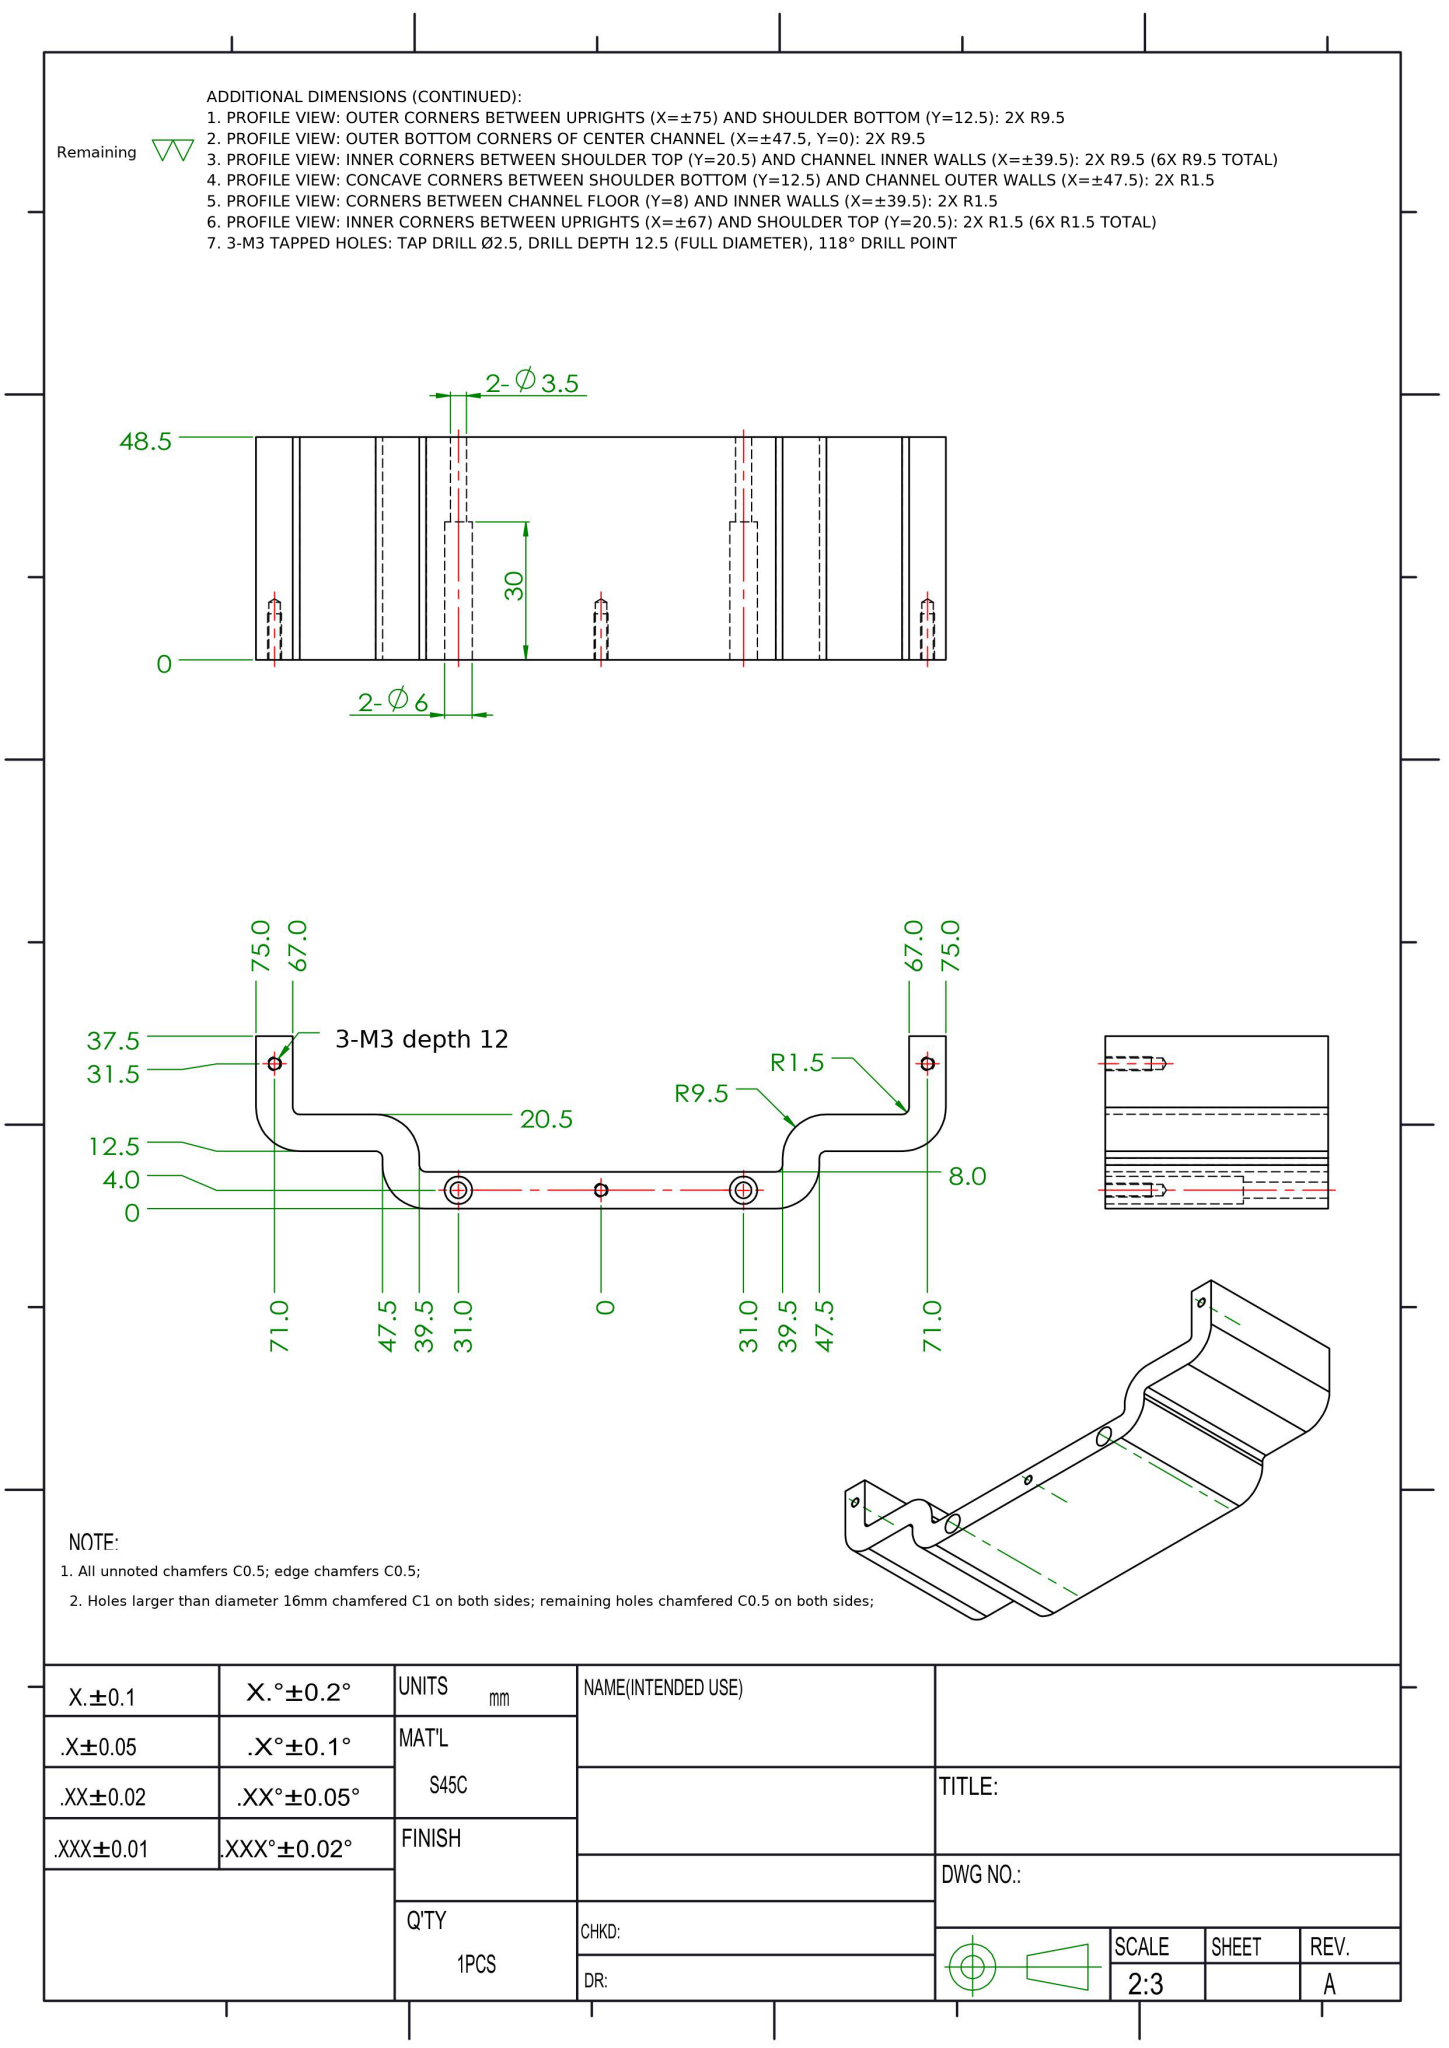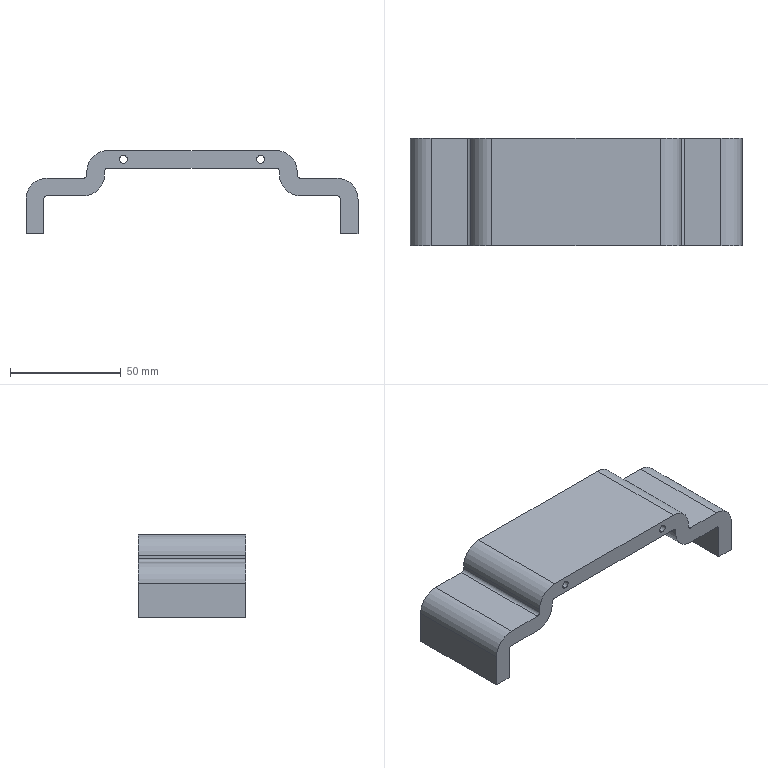Part | NX | mm | 1 solid | 52 faces | box 150 x 48.5 x 37.5 mm | volume 73356 mm3 | cylinder 26 | plane 20 | cone 6 | commonest cylinder face diameters 2.5 x6 3 x6 19 x6 6 x4 3.5 x4